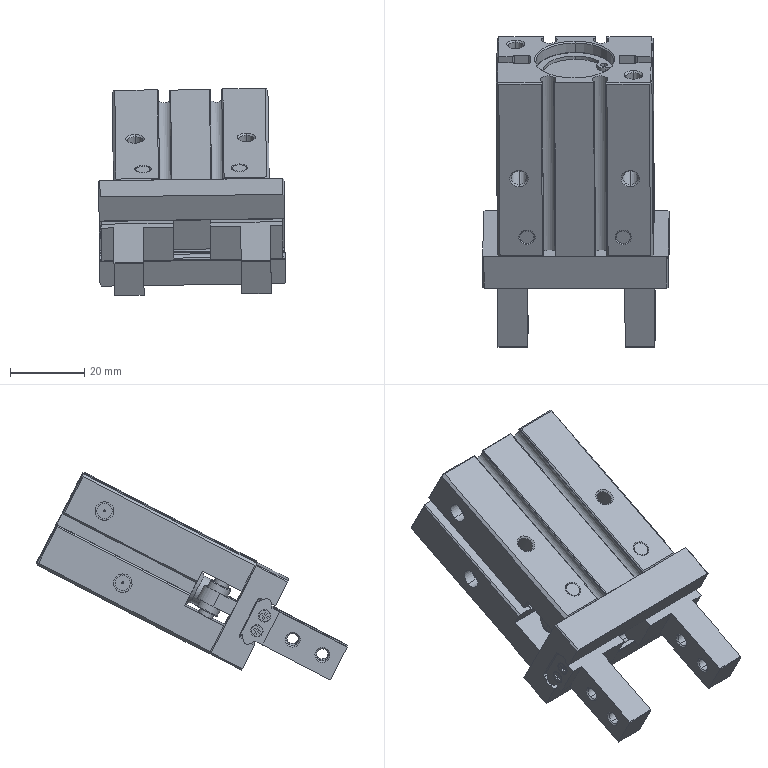Component | SolidWorks | Y0365088900012-1 | 1 solid | 459 faces | volume 63934 mm3 | plane 238 | cylinder 150 | cone 63 | spline 8 | commonest cylinder face diameters 4.134 x20 0.4 x16 4 x10 3 x10 0.8 x10 2.5 x9 6 x8 3.3 x8